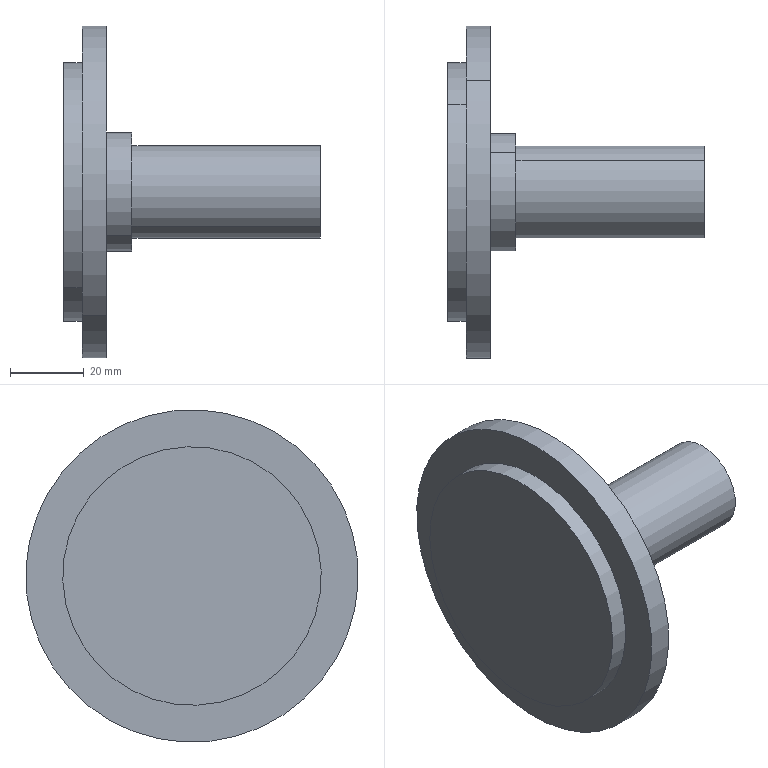Component | SolidWorks | PressurePlate-1 | 1 solid | 13 faces | box 69.5 x 90 x 90 mm | volume 91258 mm3 | cylinder 8 | plane 5 | commonest cylinder face diameters 25 x2 32 x2 70 x2 90 x2
build123d program:
from build123d import *

# Parameters (mm, degrees)
SKETCH1_R           = 45
BOSS_EXTRUDE1_DEPTH = 11.5
SKETCH16_OUTSIDE_W  = 117.56
SKETCH16_OUTSIDE_H  = 117.56
SKETCH16_OUTSIDE_R  = 35
CUT_EXTRUDE8_DEPTH  = 5
SKETCH13_R          = 16
BOSS_EXTRUDE2_DEPTH = 7
SKETCH17_R          = 12.5
BOSS_EXTRUDE3_DEPTH = 51


with BuildPart() as part:
    # Sketch1 → Boss-Extrude1 (new body)
    with BuildSketch(Plane.XY):
        Circle(SKETCH1_R)
    extrude(amount=BOSS_EXTRUDE1_DEPTH)

    # Sketch16 outside → Cut-Extrude8 (cut)
    with BuildSketch(Plane(origin=(0, 0, 0), x_dir=(-1, 0, 0), z_dir=(0, 0, -1))):
        Rectangle(SKETCH16_OUTSIDE_W, SKETCH16_OUTSIDE_H)
        Circle(SKETCH16_OUTSIDE_R, mode=Mode.SUBTRACT)
    extrude(amount=-CUT_EXTRUDE8_DEPTH, mode=Mode.SUBTRACT)

    # Sketch13 → Boss-Extrude2 (add)
    with BuildSketch(Plane.XY.offset(11.5)):
        Circle(SKETCH13_R)
    extrude(amount=BOSS_EXTRUDE2_DEPTH)

    # Sketch17 → Boss-Extrude3 (add)
    with BuildSketch(Plane.XY.offset(18.5)):
        Circle(SKETCH17_R)
    extrude(amount=BOSS_EXTRUDE3_DEPTH)


solid = part.part

# Placed as in the assembly
solid = solid.moved(Location((400.436, 1299.706, 687.116), (0, 90, 0)))
STEP:
#1=COLOUR_RGB('',0.7922,0.8196,0.9333);
#2=FILL_AREA_STYLE_COLOUR('',#1);
#3=FILL_AREA_STYLE('',(#2));
#4=SURFACE_STYLE_FILL_AREA(#3);
#5=SURFACE_SIDE_STYLE('',(#4));
#6=SURFACE_STYLE_USAGE(.BOTH.,#5);
#7=PRESENTATION_STYLE_ASSIGNMENT((#6));
#8=CARTESIAN_POINT('',(18.501,51.5,27.416));
#9=VERTEX_POINT('',#8);
#10=CARTESIAN_POINT('',(18.501,50.839,26.687));
#11=VERTEX_POINT('',#10);
#12=CARTESIAN_POINT('',(18.501,51.17,27.052));
#13=DIRECTION('',(1.,0.,0.));
#14=DIRECTION('',(-0.,0.6719,0.7406));
#15=AXIS2_PLACEMENT_3D('',#12,#13,#14);
#16=CIRCLE('',#15,0.4921);
#17=EDGE_CURVE('',#9,#11,#16,.T.);
#18=ORIENTED_EDGE('',*,*,#17,.F.);
#19=CARTESIAN_POINT('',(16.494,51.5,27.416));
#20=VERTEX_POINT('',#19);
#21=CARTESIAN_POINT('',(18.501,51.5,27.416));
#22=DIRECTION('',(-1.,-0.,-0.));
#23=VECTOR('',#22,39.37);
#24=LINE('',#21,#23);
#25=EDGE_CURVE('',#9,#20,#24,.T.);
#26=ORIENTED_EDGE('',*,*,#25,.T.);
#27=CARTESIAN_POINT('',(16.494,50.839,26.687));
#28=VERTEX_POINT('',#27);
#29=CARTESIAN_POINT('',(16.494,51.17,27.052));
#30=DIRECTION('',(1.,0.,0.));
#31=DIRECTION('',(-0.,0.6719,0.7406));
#32=AXIS2_PLACEMENT_3D('',#29,#30,#31);
#33=CIRCLE('',#32,0.4921);
#34=EDGE_CURVE('',#20,#28,#33,.T.);
#35=ORIENTED_EDGE('',*,*,#34,.T.);
#36=CARTESIAN_POINT('',(18.501,50.839,26.687));
#37=DIRECTION('',(-1.,-0.,-0.));
#38=VECTOR('',#37,39.37);
#39=LINE('',#36,#38);
#40=EDGE_CURVE('',#11,#28,#39,.T.);
#41=ORIENTED_EDGE('',*,*,#40,.F.);
#42=EDGE_LOOP('',(#18,#26,#35,#41));
#43=FACE_OUTER_BOUND('',#42,.T.);
#44=CARTESIAN_POINT('',(18.501,51.17,27.052));
#45=DIRECTION('',(-1.,-0.,-0.));
#46=DIRECTION('',(0.,-0.6719,-0.7406));
#47=AXIS2_PLACEMENT_3D('',#44,#45,#46);
#48=CYLINDRICAL_SURFACE('',#47,0.4921);
#49=ADVANCED_FACE('',(#43),#48,.T.);
#50=CARTESIAN_POINT('',(16.494,51.593,27.518));
#51=VERTEX_POINT('',#50);
#52=CARTESIAN_POINT('',(16.494,50.746,26.585));
#53=VERTEX_POINT('',#52);
#54=CARTESIAN_POINT('',(16.494,51.17,27.052));
#55=DIRECTION('',(1.,0.,0.));
#56=DIRECTION('',(-0.,0.6719,0.7406));
#57=AXIS2_PLACEMENT_3D('',#54,#55,#56);
#58=CIRCLE('',#57,0.6299);
#59=EDGE_CURVE('',#51,#53,#58,.T.);
#60=ORIENTED_EDGE('',*,*,#59,.F.);
#61=CARTESIAN_POINT('',(16.218,51.593,27.518));
#62=VERTEX_POINT('',#61);
#63=CARTESIAN_POINT('',(16.494,51.593,27.518));
#64=DIRECTION('',(-1.,-0.,-0.));
#65=VECTOR('',#64,39.37);
#66=LINE('',#63,#65);
#67=EDGE_CURVE('',#51,#62,#66,.T.);
#68=ORIENTED_EDGE('',*,*,#67,.T.);
#69=CARTESIAN_POINT('',(16.218,50.746,26.585));
#70=VERTEX_POINT('',#69);
#71=CARTESIAN_POINT('',(16.218,51.17,27.052));
#72=DIRECTION('',(1.,0.,0.));
#73=DIRECTION('',(-0.,0.6719,0.7406));
#74=AXIS2_PLACEMENT_3D('',#71,#72,#73);
#75=CIRCLE('',#74,0.6299);
#76=EDGE_CURVE('',#62,#70,#75,.T.);
#77=ORIENTED_EDGE('',*,*,#76,.T.);
#78=CARTESIAN_POINT('',(16.494,50.746,26.585));
#79=DIRECTION('',(-1.,-0.,-0.));
#80=VECTOR('',#79,39.37);
#81=LINE('',#78,#80);
#82=EDGE_CURVE('',#53,#70,#81,.T.);
#83=ORIENTED_EDGE('',*,*,#82,.F.);
#84=EDGE_LOOP('',(#60,#68,#77,#83));
#85=FACE_OUTER_BOUND('',#84,.T.);
#86=CARTESIAN_POINT('',(16.494,51.17,27.052));
#87=DIRECTION('',(-1.,-0.,-0.));
#88=DIRECTION('',(0.,-0.6719,-0.7406));
#89=AXIS2_PLACEMENT_3D('',#86,#87,#88);
#90=CYLINDRICAL_SURFACE('',#89,0.6299);
#91=ADVANCED_FACE('',(#85),#90,.T.);
#92=CARTESIAN_POINT('',(15.962,50.244,26.031));
#93=VERTEX_POINT('',#92);
#94=CARTESIAN_POINT('',(15.962,52.095,28.072));
#95=VERTEX_POINT('',#94);
#96=CARTESIAN_POINT('',(15.962,51.17,27.052));
#97=DIRECTION('',(-1.,-0.,-0.));
#98=DIRECTION('',(0.,-0.6719,-0.7406));
#99=AXIS2_PLACEMENT_3D('',#96,#97,#98);
#100=CIRCLE('',#99,1.378);
#101=EDGE_CURVE('',#93,#95,#100,.T.);
#102=ORIENTED_EDGE('',*,*,#101,.T.);
#103=CARTESIAN_POINT('',(15.765,52.095,28.072));
#104=VERTEX_POINT('',#103);
#105=CARTESIAN_POINT('',(15.962,52.095,28.072));
#106=DIRECTION('',(-1.,-0.,-0.));
#107=VECTOR('',#106,39.37);
#108=LINE('',#105,#107);
#109=EDGE_CURVE('',#95,#104,#108,.T.);
#110=ORIENTED_EDGE('',*,*,#109,.T.);
#111=CARTESIAN_POINT('',(15.765,50.244,26.031));
#112=VERTEX_POINT('',#111);
#113=CARTESIAN_POINT('',(15.765,51.17,27.052));
#114=DIRECTION('',(-1.,-0.,-0.));
#115=DIRECTION('',(0.,-0.6719,-0.7406));
#116=AXIS2_PLACEMENT_3D('',#113,#114,#115);
#117=CIRCLE('',#116,1.378);
#118=EDGE_CURVE('',#112,#104,#117,.T.);
#119=ORIENTED_EDGE('',*,*,#118,.F.);
#120=CARTESIAN_POINT('',(15.962,50.244,26.031));
#121=DIRECTION('',(-1.,-0.,-0.));
#122=VECTOR('',#121,39.37);
#123=LINE('',#120,#122);
#124=EDGE_CURVE('',#93,#112,#123,.T.);
#125=ORIENTED_EDGE('',*,*,#124,.F.);
#126=EDGE_LOOP('',(#102,#110,#119,#125));
#127=FACE_OUTER_BOUND('',#126,.T.);
#128=CARTESIAN_POINT('',(15.962,51.17,27.052));
#129=DIRECTION('',(-1.,-0.,-0.));
#130=DIRECTION('',(0.,-0.6719,-0.7406));
#131=AXIS2_PLACEMENT_3D('',#128,#129,#130);
#132=CYLINDRICAL_SURFACE('',#131,1.378);
#133=ADVANCED_FACE('',(#127),#132,.T.);
#134=CARTESIAN_POINT('',(16.218,52.36,28.364));
#135=VERTEX_POINT('',#134);
#136=CARTESIAN_POINT('',(16.218,49.979,25.74));
#137=VERTEX_POINT('',#136);
#138=CARTESIAN_POINT('',(16.218,51.17,27.052));
#139=DIRECTION('',(1.,0.,0.));
#140=DIRECTION('',(-0.,0.6719,0.7406));
#141=AXIS2_PLACEMENT_3D('',#138,#139,#140);
#142=CIRCLE('',#141,1.772);
#143=EDGE_CURVE('',#135,#137,#142,.T.);
#144=ORIENTED_EDGE('',*,*,#143,.F.);
#145=CARTESIAN_POINT('',(15.962,52.36,28.364));
#146=VERTEX_POINT('',#145);
#147=CARTESIAN_POINT('',(16.218,52.36,28.364));
#148=DIRECTION('',(-1.,-0.,-0.));
#149=VECTOR('',#148,39.37);
#150=LINE('',#147,#149);
#151=EDGE_CURVE('',#135,#146,#150,.T.);
#152=ORIENTED_EDGE('',*,*,#151,.T.);
#153=CARTESIAN_POINT('',(15.962,49.979,25.74));
#154=VERTEX_POINT('',#153);
#155=CARTESIAN_POINT('',(15.962,51.17,27.052));
#156=DIRECTION('',(-1.,-0.,-0.));
#157=DIRECTION('',(0.,-0.6719,-0.7406));
#158=AXIS2_PLACEMENT_3D('',#155,#156,#157);
#159=CIRCLE('',#158,1.772);
#160=EDGE_CURVE('',#154,#146,#159,.T.);
#161=ORIENTED_EDGE('',*,*,#160,.F.);
#162=CARTESIAN_POINT('',(16.218,49.979,25.74));
#163=DIRECTION('',(-1.,-0.,-0.));
#164=VECTOR('',#163,39.37);
#165=LINE('',#162,#164);
#166=EDGE_CURVE('',#137,#154,#165,.T.);
#167=ORIENTED_EDGE('',*,*,#166,.F.);
#168=EDGE_LOOP('',(#144,#152,#161,#167));
#169=FACE_OUTER_BOUND('',#168,.T.);
#170=CARTESIAN_POINT('',(16.218,51.17,27.052));
#171=DIRECTION('',(-1.,-0.,-0.));
#172=DIRECTION('',(0.,-0.6719,-0.7406));
#173=AXIS2_PLACEMENT_3D('',#170,#171,#172);
#174=CYLINDRICAL_SURFACE('',#173,1.772);
#175=ADVANCED_FACE('',(#169),#174,.T.);
#176=ORIENTED_EDGE('',*,*,#151,.F.);
#177=CARTESIAN_POINT('',(16.218,51.17,27.052));
#178=DIRECTION('',(1.,0.,0.));
#179=DIRECTION('',(-0.,0.6719,0.7406));
#180=AXIS2_PLACEMENT_3D('',#177,#178,#179);
#181=CIRCLE('',#180,1.772);
#182=EDGE_CURVE('',#137,#135,#181,.T.);
#183=ORIENTED_EDGE('',*,*,#182,.F.);
#184=ORIENTED_EDGE('',*,*,#166,.T.);
#185=CARTESIAN_POINT('',(15.962,51.17,27.052));
#186=DIRECTION('',(-1.,-0.,-0.));
#187=DIRECTION('',(0.,-0.6719,-0.7406));
#188=AXIS2_PLACEMENT_3D('',#185,#186,#187);
#189=CIRCLE('',#188,1.772);
#190=EDGE_CURVE('',#146,#154,#189,.T.);
#191=ORIENTED_EDGE('',*,*,#190,.F.);
#192=EDGE_LOOP('',(#176,#183,#184,#191));
#193=FACE_OUTER_BOUND('',#192,.T.);
#194=CARTESIAN_POINT('',(16.218,51.17,27.052));
#195=DIRECTION('',(-1.,-0.,-0.));
#196=DIRECTION('',(0.,-0.6719,-0.7406));
#197=AXIS2_PLACEMENT_3D('',#194,#195,#196);
#198=CYLINDRICAL_SURFACE('',#197,1.772);
#199=ADVANCED_FACE('',(#193),#198,.T.);
#200=CARTESIAN_POINT('',(16.218,51.17,27.052));
#201=DIRECTION('',(1.,0.,0.));
#202=DIRECTION('',(-0.,0.6719,0.7406));
#203=AXIS2_PLACEMENT_3D('',#200,#201,#202);
#204=CIRCLE('',#203,0.6299);
#205=EDGE_CURVE('',#70,#62,#204,.T.);
#206=ORIENTED_EDGE('',*,*,#205,.F.);
#207=ORIENTED_EDGE('',*,*,#76,.F.);
#208=EDGE_LOOP('',(#206,#207));
#209=FACE_BOUND('',#208,.T.);
#210=ORIENTED_EDGE('',*,*,#182,.T.);
#211=ORIENTED_EDGE('',*,*,#143,.T.);
#212=EDGE_LOOP('',(#210,#211));
#213=FACE_OUTER_BOUND('',#212,.T.);
#214=CARTESIAN_POINT('',(16.218,51.17,27.052));
#215=DIRECTION('',(1.,0.,0.));
#216=DIRECTION('',(-0.,0.6719,0.7406));
#217=AXIS2_PLACEMENT_3D('',#214,#215,#216);
#218=PLANE('',#217);
#219=ADVANCED_FACE('',(#209,#213),#218,.T.);
#220=ORIENTED_EDGE('',*,*,#101,.F.);
#221=CARTESIAN_POINT('',(15.962,51.17,27.052));
#222=DIRECTION('',(-1.,-0.,-0.));
#223=DIRECTION('',(0.,-0.6719,-0.7406));
#224=AXIS2_PLACEMENT_3D('',#221,#222,#223);
#225=CIRCLE('',#224,1.378);
#226=EDGE_CURVE('',#95,#93,#225,.T.);
#227=ORIENTED_EDGE('',*,*,#226,.F.);
#228=EDGE_LOOP('',(#220,#227));
#229=FACE_BOUND('',#228,.T.);
#230=ORIENTED_EDGE('',*,*,#160,.T.);
#231=ORIENTED_EDGE('',*,*,#190,.T.);
#232=EDGE_LOOP('',(#230,#231));
#233=FACE_OUTER_BOUND('',#232,.T.);
#234=CARTESIAN_POINT('',(15.962,51.17,27.052));
#235=DIRECTION('',(-1.,-0.,-0.));
#236=DIRECTION('',(0.,-0.6719,-0.7406));
#237=AXIS2_PLACEMENT_3D('',#234,#235,#236);
#238=PLANE('',#237);
#239=ADVANCED_FACE('',(#229,#233),#238,.T.);
#240=ORIENTED_EDGE('',*,*,#109,.F.);
#241=ORIENTED_EDGE('',*,*,#226,.T.);
#242=ORIENTED_EDGE('',*,*,#124,.T.);
#243=CARTESIAN_POINT('',(15.765,51.17,27.052));
#244=DIRECTION('',(-1.,-0.,-0.));
#245=DIRECTION('',(0.,-0.6719,-0.7406));
#246=AXIS2_PLACEMENT_3D('',#243,#244,#245);
#247=CIRCLE('',#246,1.378);
#248=EDGE_CURVE('',#104,#112,#247,.T.);
#249=ORIENTED_EDGE('',*,*,#248,.F.);
#250=EDGE_LOOP('',(#240,#241,#242,#249));
#251=FACE_OUTER_BOUND('',#250,.T.);
#252=CARTESIAN_POINT('',(15.962,51.17,27.052));
#253=DIRECTION('',(-1.,-0.,-0.));
#254=DIRECTION('',(0.,-0.6719,-0.7406));
#255=AXIS2_PLACEMENT_3D('',#252,#253,#254);
#256=CYLINDRICAL_SURFACE('',#255,1.378);
#257=ADVANCED_FACE('',(#251),#256,.T.);
#258=ORIENTED_EDGE('',*,*,#118,.T.);
#259=ORIENTED_EDGE('',*,*,#248,.T.);
#260=EDGE_LOOP('',(#258,#259));
#261=FACE_OUTER_BOUND('',#260,.T.);
#262=CARTESIAN_POINT('',(15.765,51.17,27.052));
#263=DIRECTION('',(1.,0.,0.));
#264=DIRECTION('',(-0.,0.6719,0.7406));
#265=AXIS2_PLACEMENT_3D('',#262,#263,#264);
#266=PLANE('',#265);
#267=ADVANCED_FACE('',(#261),#266,.F.);
#268=ORIENTED_EDGE('',*,*,#67,.F.);
#269=CARTESIAN_POINT('',(16.494,51.17,27.052));
#270=DIRECTION('',(1.,0.,0.));
#271=DIRECTION('',(-0.,0.6719,0.7406));
#272=AXIS2_PLACEMENT_3D('',#269,#270,#271);
#273=CIRCLE('',#272,0.6299);
#274=EDGE_CURVE('',#53,#51,#273,.T.);
#275=ORIENTED_EDGE('',*,*,#274,.F.);
#276=ORIENTED_EDGE('',*,*,#82,.T.);
#277=ORIENTED_EDGE('',*,*,#205,.T.);
#278=EDGE_LOOP('',(#268,#275,#276,#277));
#279=FACE_OUTER_BOUND('',#278,.T.);
#280=CARTESIAN_POINT('',(16.494,51.17,27.052));
#281=DIRECTION('',(-1.,-0.,-0.));
#282=DIRECTION('',(0.,-0.6719,-0.7406));
#283=AXIS2_PLACEMENT_3D('',#280,#281,#282);
#284=CYLINDRICAL_SURFACE('',#283,0.6299);
#285=ADVANCED_FACE('',(#279),#284,.T.);
#286=CARTESIAN_POINT('',(16.494,51.17,27.052));
#287=DIRECTION('',(1.,0.,0.));
#288=DIRECTION('',(-0.,0.6719,0.7406));
#289=AXIS2_PLACEMENT_3D('',#286,#287,#288);
#290=CIRCLE('',#289,0.4921);
#291=EDGE_CURVE('',#28,#20,#290,.T.);
#292=ORIENTED_EDGE('',*,*,#291,.F.);
#293=ORIENTED_EDGE('',*,*,#34,.F.);
#294=EDGE_LOOP('',(#292,#293));
#295=FACE_BOUND('',#294,.T.);
#296=ORIENTED_EDGE('',*,*,#274,.T.);
#297=ORIENTED_EDGE('',*,*,#59,.T.);
#298=EDGE_LOOP('',(#296,#297));
#299=FACE_OUTER_BOUND('',#298,.T.);
#300=CARTESIAN_POINT('',(16.494,51.17,27.052));
#301=DIRECTION('',(1.,0.,0.));
#302=DIRECTION('',(-0.,0.6719,0.7406));
#303=AXIS2_PLACEMENT_3D('',#300,#301,#302);
#304=PLANE('',#303);
#305=ADVANCED_FACE('',(#295,#299),#304,.T.);
#306=ORIENTED_EDGE('',*,*,#25,.F.);
#307=CARTESIAN_POINT('',(18.501,51.17,27.052));
#308=DIRECTION('',(1.,0.,0.));
#309=DIRECTION('',(-0.,0.6719,0.7406));
#310=AXIS2_PLACEMENT_3D('',#307,#308,#309);
#311=CIRCLE('',#310,0.4921);
#312=EDGE_CURVE('',#11,#9,#311,.T.);
#313=ORIENTED_EDGE('',*,*,#312,.F.);
#314=ORIENTED_EDGE('',*,*,#40,.T.);
#315=ORIENTED_EDGE('',*,*,#291,.T.);
#316=EDGE_LOOP('',(#306,#313,#314,#315));
#317=FACE_OUTER_BOUND('',#316,.T.);
#318=CARTESIAN_POINT('',(18.501,51.17,27.052));
#319=DIRECTION('',(-1.,-0.,-0.));
#320=DIRECTION('',(0.,-0.6719,-0.7406));
#321=AXIS2_PLACEMENT_3D('',#318,#319,#320);
#322=CYLINDRICAL_SURFACE('',#321,0.4921);
#323=ADVANCED_FACE('',(#317),#322,.T.);
#324=ORIENTED_EDGE('',*,*,#312,.T.);
#325=ORIENTED_EDGE('',*,*,#17,.T.);
#326=EDGE_LOOP('',(#324,#325));
#327=FACE_OUTER_BOUND('',#326,.T.);
#328=CARTESIAN_POINT('',(18.501,51.17,27.052));
#329=DIRECTION('',(1.,0.,0.));
#330=DIRECTION('',(-0.,0.6719,0.7406));
#331=AXIS2_PLACEMENT_3D('',#328,#329,#330);
#332=PLANE('',#331);
#333=ADVANCED_FACE('',(#327),#332,.T.);
#334=CLOSED_SHELL('',(#49,#91,#133,#175,#199,#219,#239,#257,#267,#285,#305,#323,#333));
#335=MANIFOLD_SOLID_BREP('',#334);
#336=STYLED_ITEM('',(#7),#335);
#337=(LENGTH_UNIT()NAMED_UNIT(*)SI_UNIT($,.METRE.));
#338=LENGTH_MEASURE_WITH_UNIT(LENGTH_MEASURE(0.0254),#337);
#339=DIMENSIONAL_EXPONENTS(1.,0.,0.,0.,0.,0.,0.);
#340=(CONVERSION_BASED_UNIT('',#338)LENGTH_UNIT()NAMED_UNIT(#339));
#341=UNCERTAINTY_MEASURE_WITH_UNIT(LENGTH_MEASURE(0.00001),#340,'','');
#342=(NAMED_UNIT(*)PLANE_ANGLE_UNIT()SI_UNIT($,.RADIAN.));
#343=(NAMED_UNIT(*)SI_UNIT($,.STERADIAN.)SOLID_ANGLE_UNIT());
#344=(GEOMETRIC_REPRESENTATION_CONTEXT(3)GLOBAL_UNCERTAINTY_ASSIGNED_CONTEXT((#341))GLOBAL_UNIT_ASSIGNED_CONTEXT((#340,#342,#343))REPRESENTATION_CONTEXT('',''));
#345=MECHANICAL_DESIGN_GEOMETRIC_PRESENTATION_REPRESENTATION('',(#336),#344);
#346=PRESENTATION_LAYER_ASSIGNMENT('','',(#336));
#347=CARTESIAN_POINT('',(0.,0.,0.));
#348=DIRECTION('',(0.,0.,1.));
#349=DIRECTION('',(1.,0.,0.));
#350=AXIS2_PLACEMENT_3D('',#347,#348,#349);
#351=(LENGTH_UNIT()NAMED_UNIT(*)SI_UNIT($,.METRE.));
#352=LENGTH_MEASURE_WITH_UNIT(LENGTH_MEASURE(0.0254),#351);
#353=DIMENSIONAL_EXPONENTS(1.,0.,0.,0.,0.,0.,0.);
#354=(CONVERSION_BASED_UNIT('',#352)LENGTH_UNIT()NAMED_UNIT(#353));
#355=UNCERTAINTY_MEASURE_WITH_UNIT(LENGTH_MEASURE(0.00001),#354,'','');
#356=(NAMED_UNIT(*)PLANE_ANGLE_UNIT()SI_UNIT($,.RADIAN.));
#357=(NAMED_UNIT(*)SI_UNIT($,.STERADIAN.)SOLID_ANGLE_UNIT());
#358=(GEOMETRIC_REPRESENTATION_CONTEXT(3)GLOBAL_UNCERTAINTY_ASSIGNED_CONTEXT((#355))GLOBAL_UNIT_ASSIGNED_CONTEXT((#354,#356,#357))REPRESENTATION_CONTEXT('',''));
#359=ADVANCED_BREP_SHAPE_REPRESENTATION('',(#335,#350),#358);